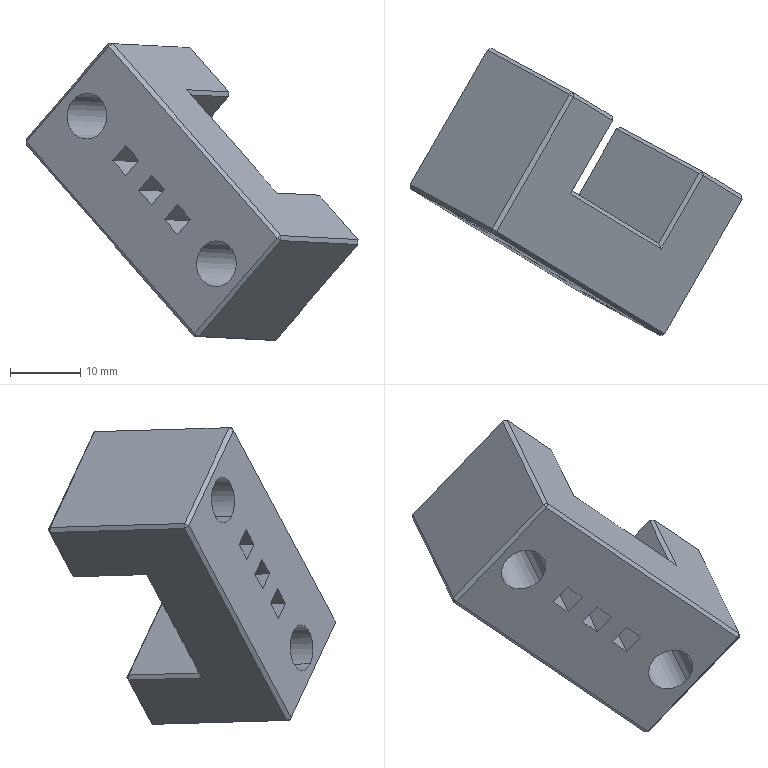Component | SolidWorks | 4z0-123-1 | 1 solid | 66 faces | box 47.11 x 40.74 x 42.09 mm | volume 12284 mm3 | plane 58 | cylinder 8 | commonest cylinder face diameters 6.5 x4 3.4 x4
build123d program:
from build123d import *

# Parameters (mm, degrees)
SKETCH1_W                                       = 40
SKETCH1_H                                       = 20
BOSS_EXTRUDE1_DEPTH                             = 23
SKETCH2_W                                       = 3
SKETCH2_H                                       = 3
CUT_EXTRUDE1_DEPTH                              = 33.078
LPATTERN1_COUNT                                 = 2
LPATTERN1_PITCH                                 = 6
LPATTERN2_COUNT                                 = 2
LPATTERN2_PITCH                                 = 6
M3_HEX_SOCKET_HEAD_CAP_SCREW_CBORE1_D           = 3.4
M3_HEX_SOCKET_HEAD_CAP_SCREW_CBORE1_CBORE_D     = 6.5
M3_HEX_SOCKET_HEAD_CAP_SCREW_CBORE1_CBORE_DEPTH = 11.4
SKETCH7_W                                       = 20
SKETCH7_H                                       = 24
CUT_EXTRUDE2_DEPTH                              = 37.455
CHAMFER1_SIZE                                   = 0.5


with BuildPart() as part:
    # Sketch1 → Boss-Extrude1 (new body)
    with BuildSketch(Plane.XY):
        Rectangle(SKETCH1_W, SKETCH1_H)
    extrude(amount=BOSS_EXTRUDE1_DEPTH)

    # Sketch2 → Cut-Extrude1 (cut, through all)
    with BuildSketch(Plane.XY.offset(23)):
        Rectangle(SKETCH2_W, SKETCH2_H)
    cut_extrude1 = extrude(amount=-CUT_EXTRUDE1_DEPTH, mode=Mode.SUBTRACT)

    # LPattern1: Cut-Extrude1 ×2
    with Locations(*[(i * LPATTERN1_PITCH, 0, 0) for i in range(1, LPATTERN1_COUNT)]):
        add(cut_extrude1, mode=Mode.SUBTRACT)

    # LPattern2: Cut-Extrude1 ×2
    with Locations(*[(-i * LPATTERN2_PITCH, 0, 0) for i in range(1, LPATTERN2_COUNT)]):
        add(cut_extrude1, mode=Mode.SUBTRACT)

    # M3 Hex Socket Head Cap Screw CBORE1 (through all)
    with Locations(Plane.XY.offset(23)):
        with Locations((-15, 0), (15, 0)):
            CounterBoreHole(M3_HEX_SOCKET_HEAD_CAP_SCREW_CBORE1_D / 2, M3_HEX_SOCKET_HEAD_CAP_SCREW_CBORE1_CBORE_D / 2, M3_HEX_SOCKET_HEAD_CAP_SCREW_CBORE1_CBORE_DEPTH)

    # Sketch7 → Cut-Extrude2 (cut, through all)
    with BuildSketch(Plane.XZ.offset(10)):
        Rectangle(SKETCH7_W, SKETCH7_H)
    extrude(amount=-CUT_EXTRUDE2_DEPTH, mode=Mode.SUBTRACT)

    # Chamfer1
    chamfer1_edges = [part.edges().sort_by_distance(p)[0] for p in [
        (-20, 0, 23),
        (0, -10, 23),
        (20, 0, 23),
        (-15, -10, 0),
        (-20, 0, 0),
        (15, 10, 0),
        (20, 0, 0),
        (0, 10, 23),
        (20, -10, 11.5),
        (-20, -10, 11.5),
        (-20, 10, 11.5),
        (20, 10, 11.5),
        (15, -10, 0),
        (-15, 10, 0),
        (-10, 0, 0),
        (10, 0, 0),
        (10, 10, 6),
        (-10, 10, 6),
        (-10, -10, 6),
        (10, -10, 6),
        (0, -10, 12),
        (0, 10, 12),
    ]]
    chamfer(chamfer1_edges, length=CHAMFER1_SIZE)


solid = part.part

# Placed as in the assembly
solid = solid.moved(Location((-78.851, -91.285, 77.48), (88.336, -29.849, 134.87)))